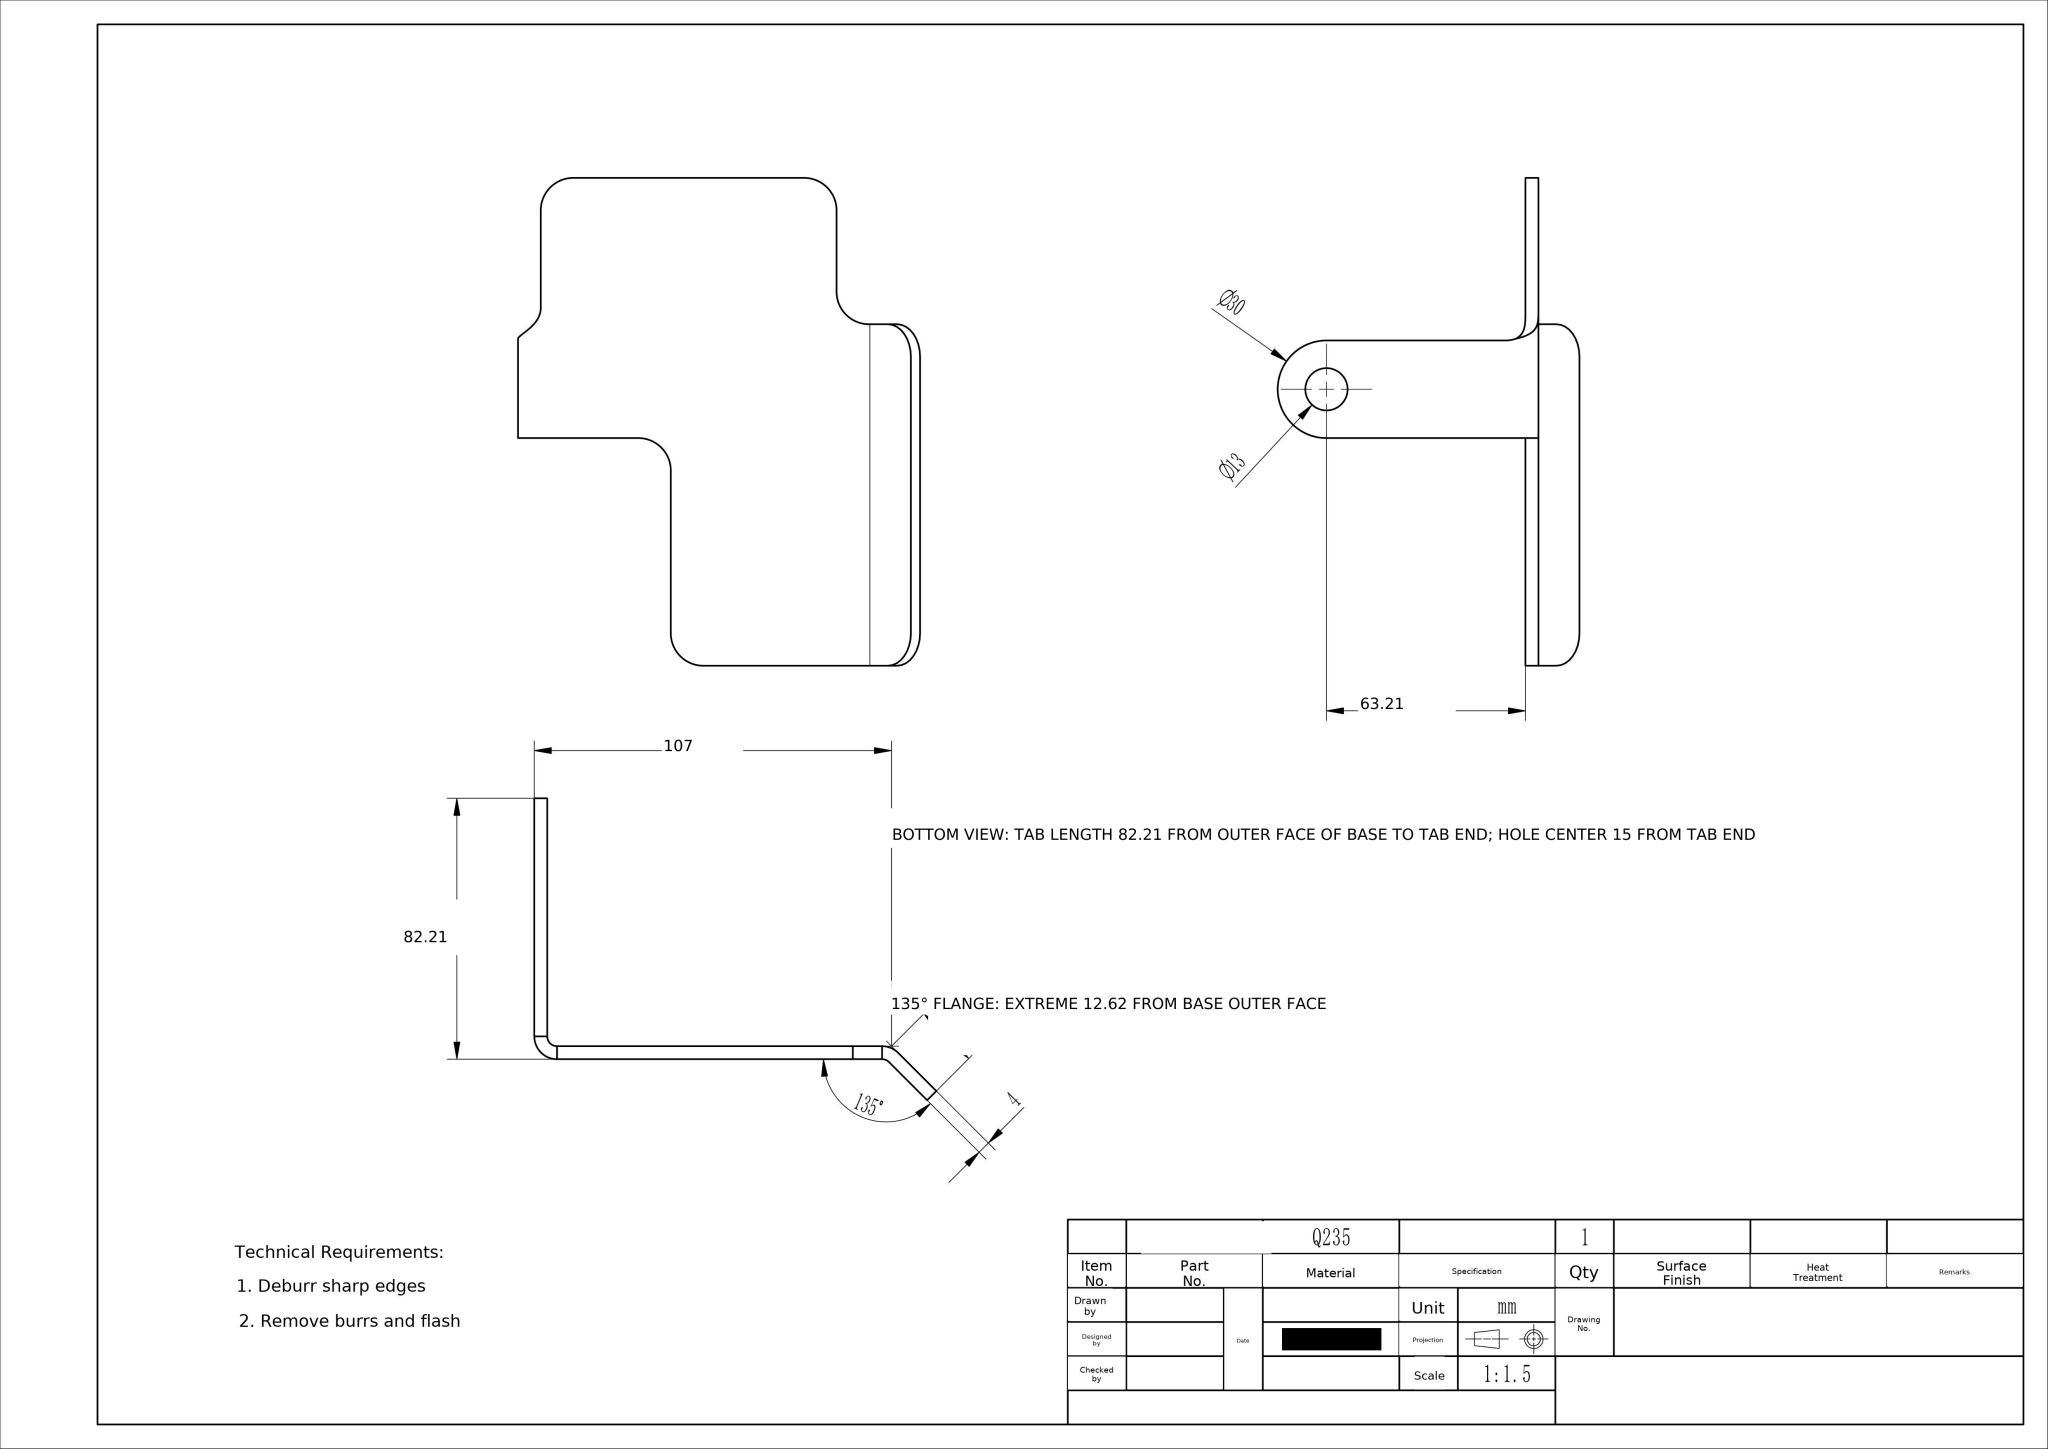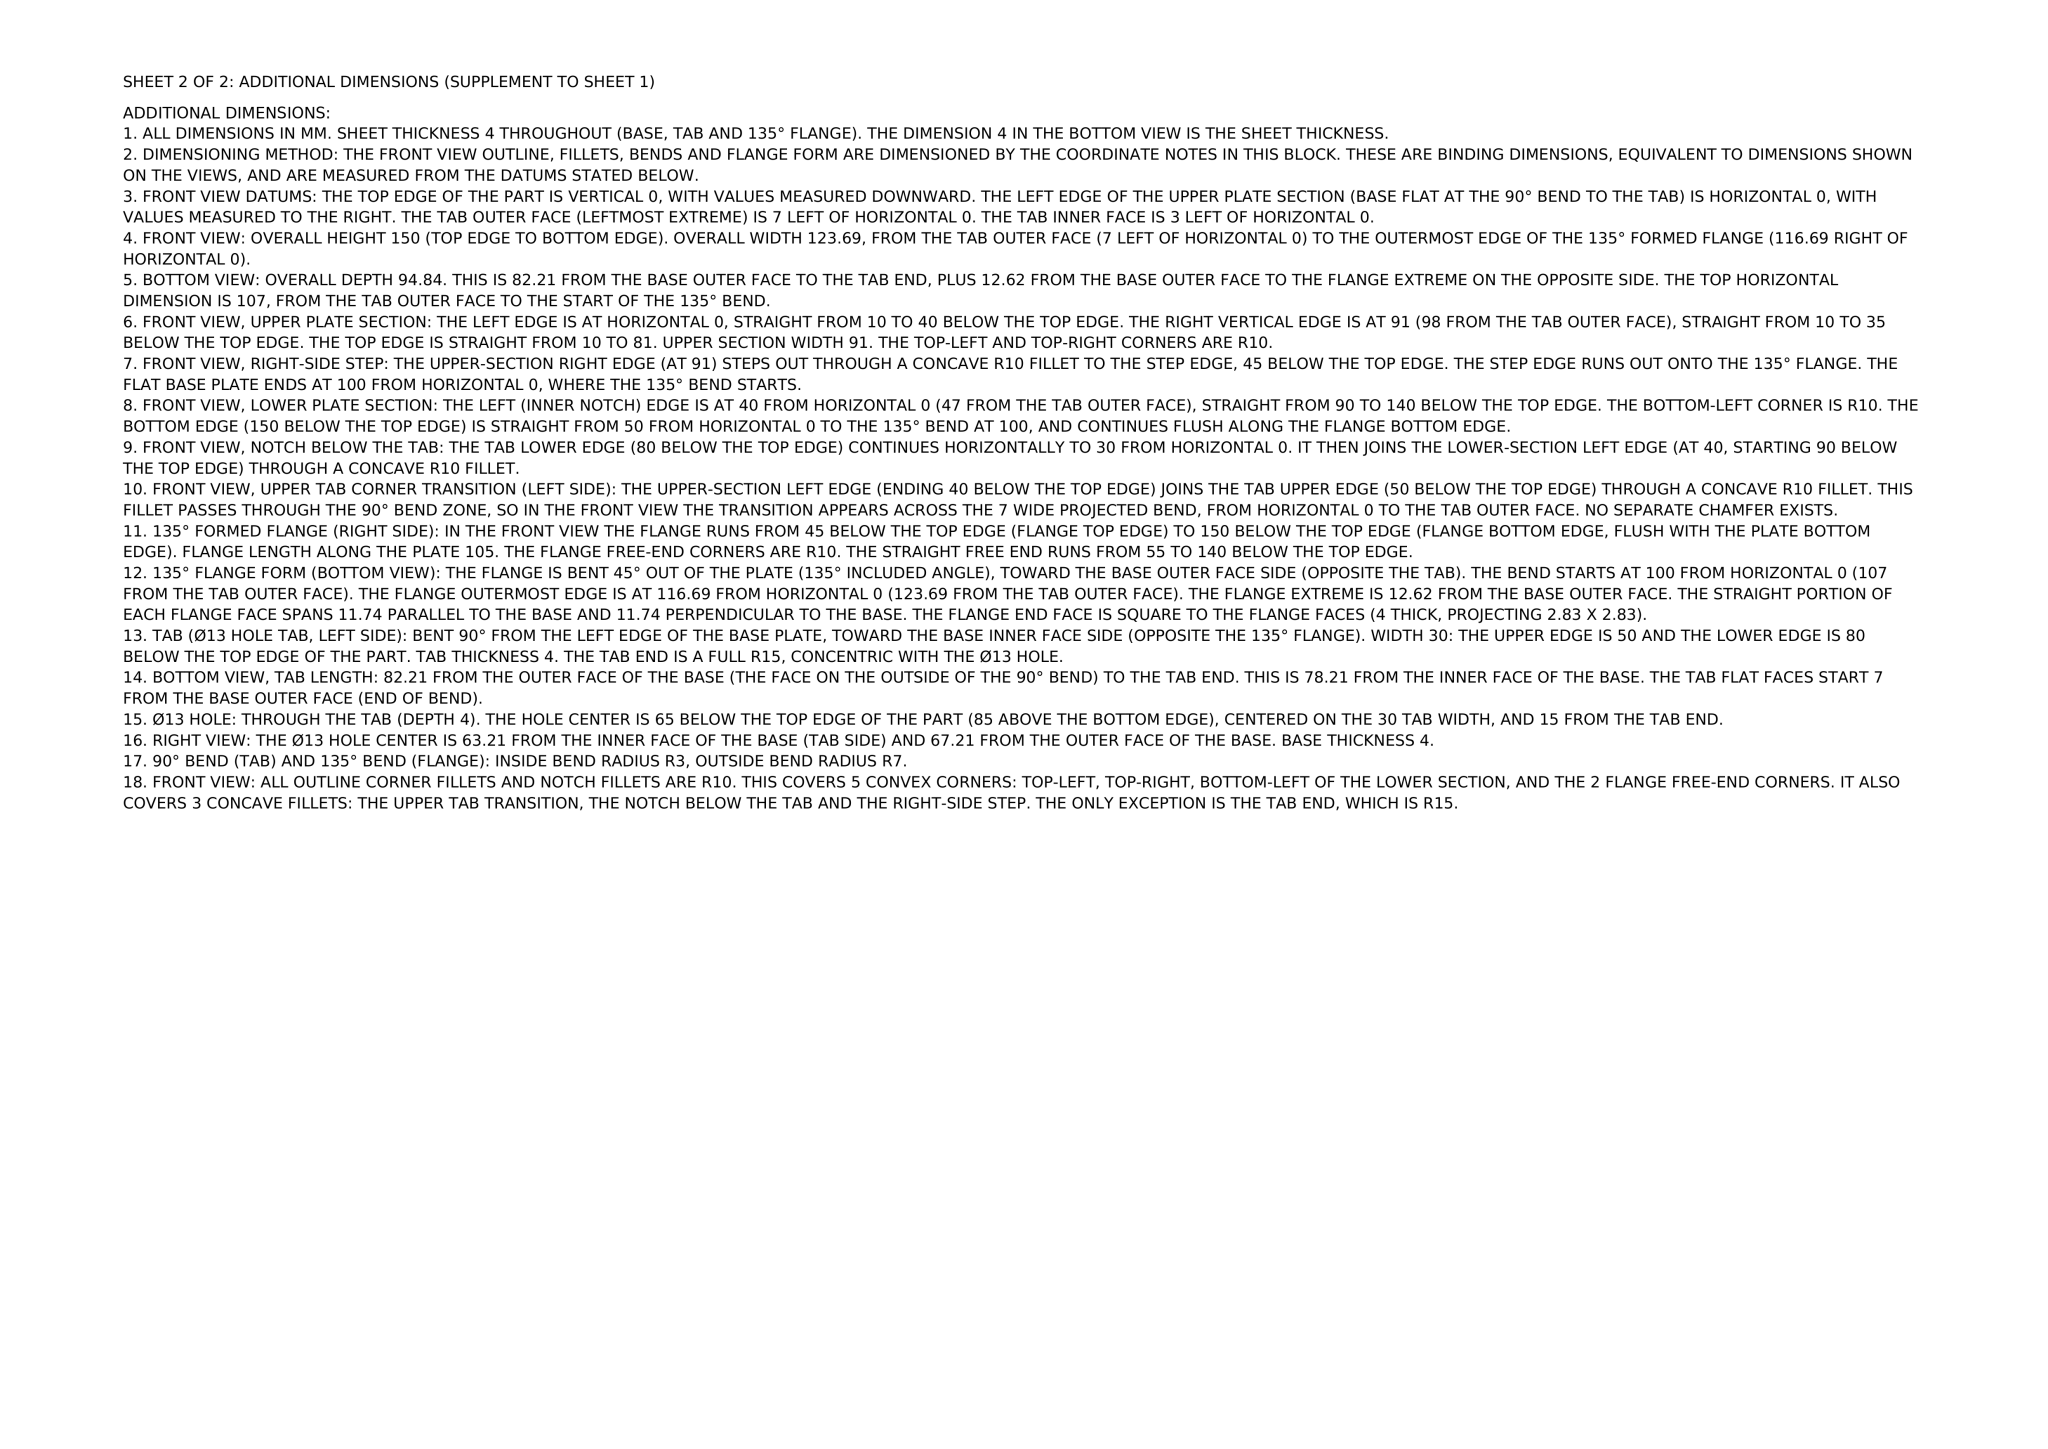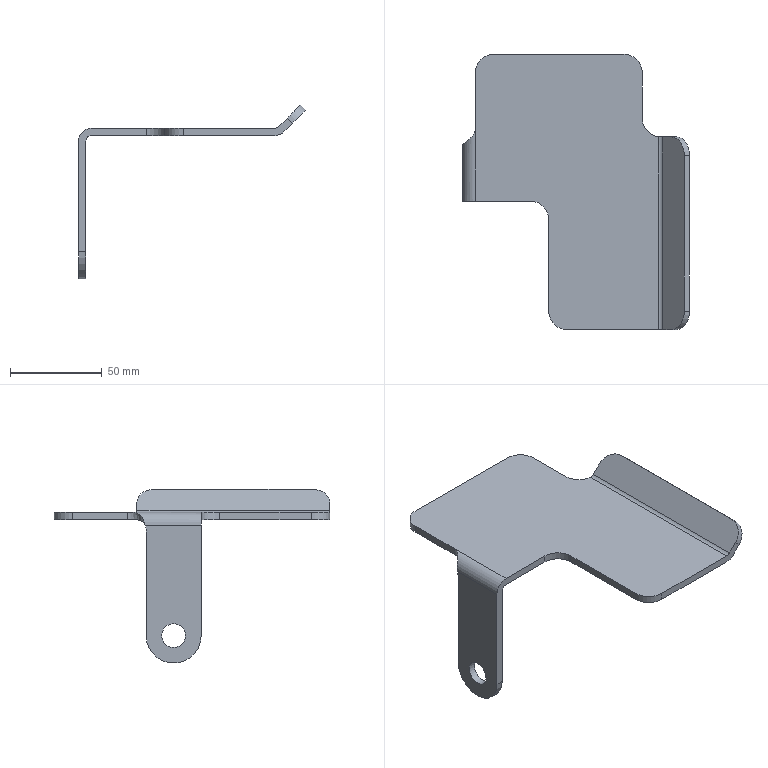Part | NX | mm | 1 solid | 31 faces | box 123.69 x 150 x 94.84 mm | volume 64697 mm3 | plane 15 | cylinder 14 | spline 2 | commonest cylinder face diameters 20 x8 14 x2 6 x2 30 x1 13 x1